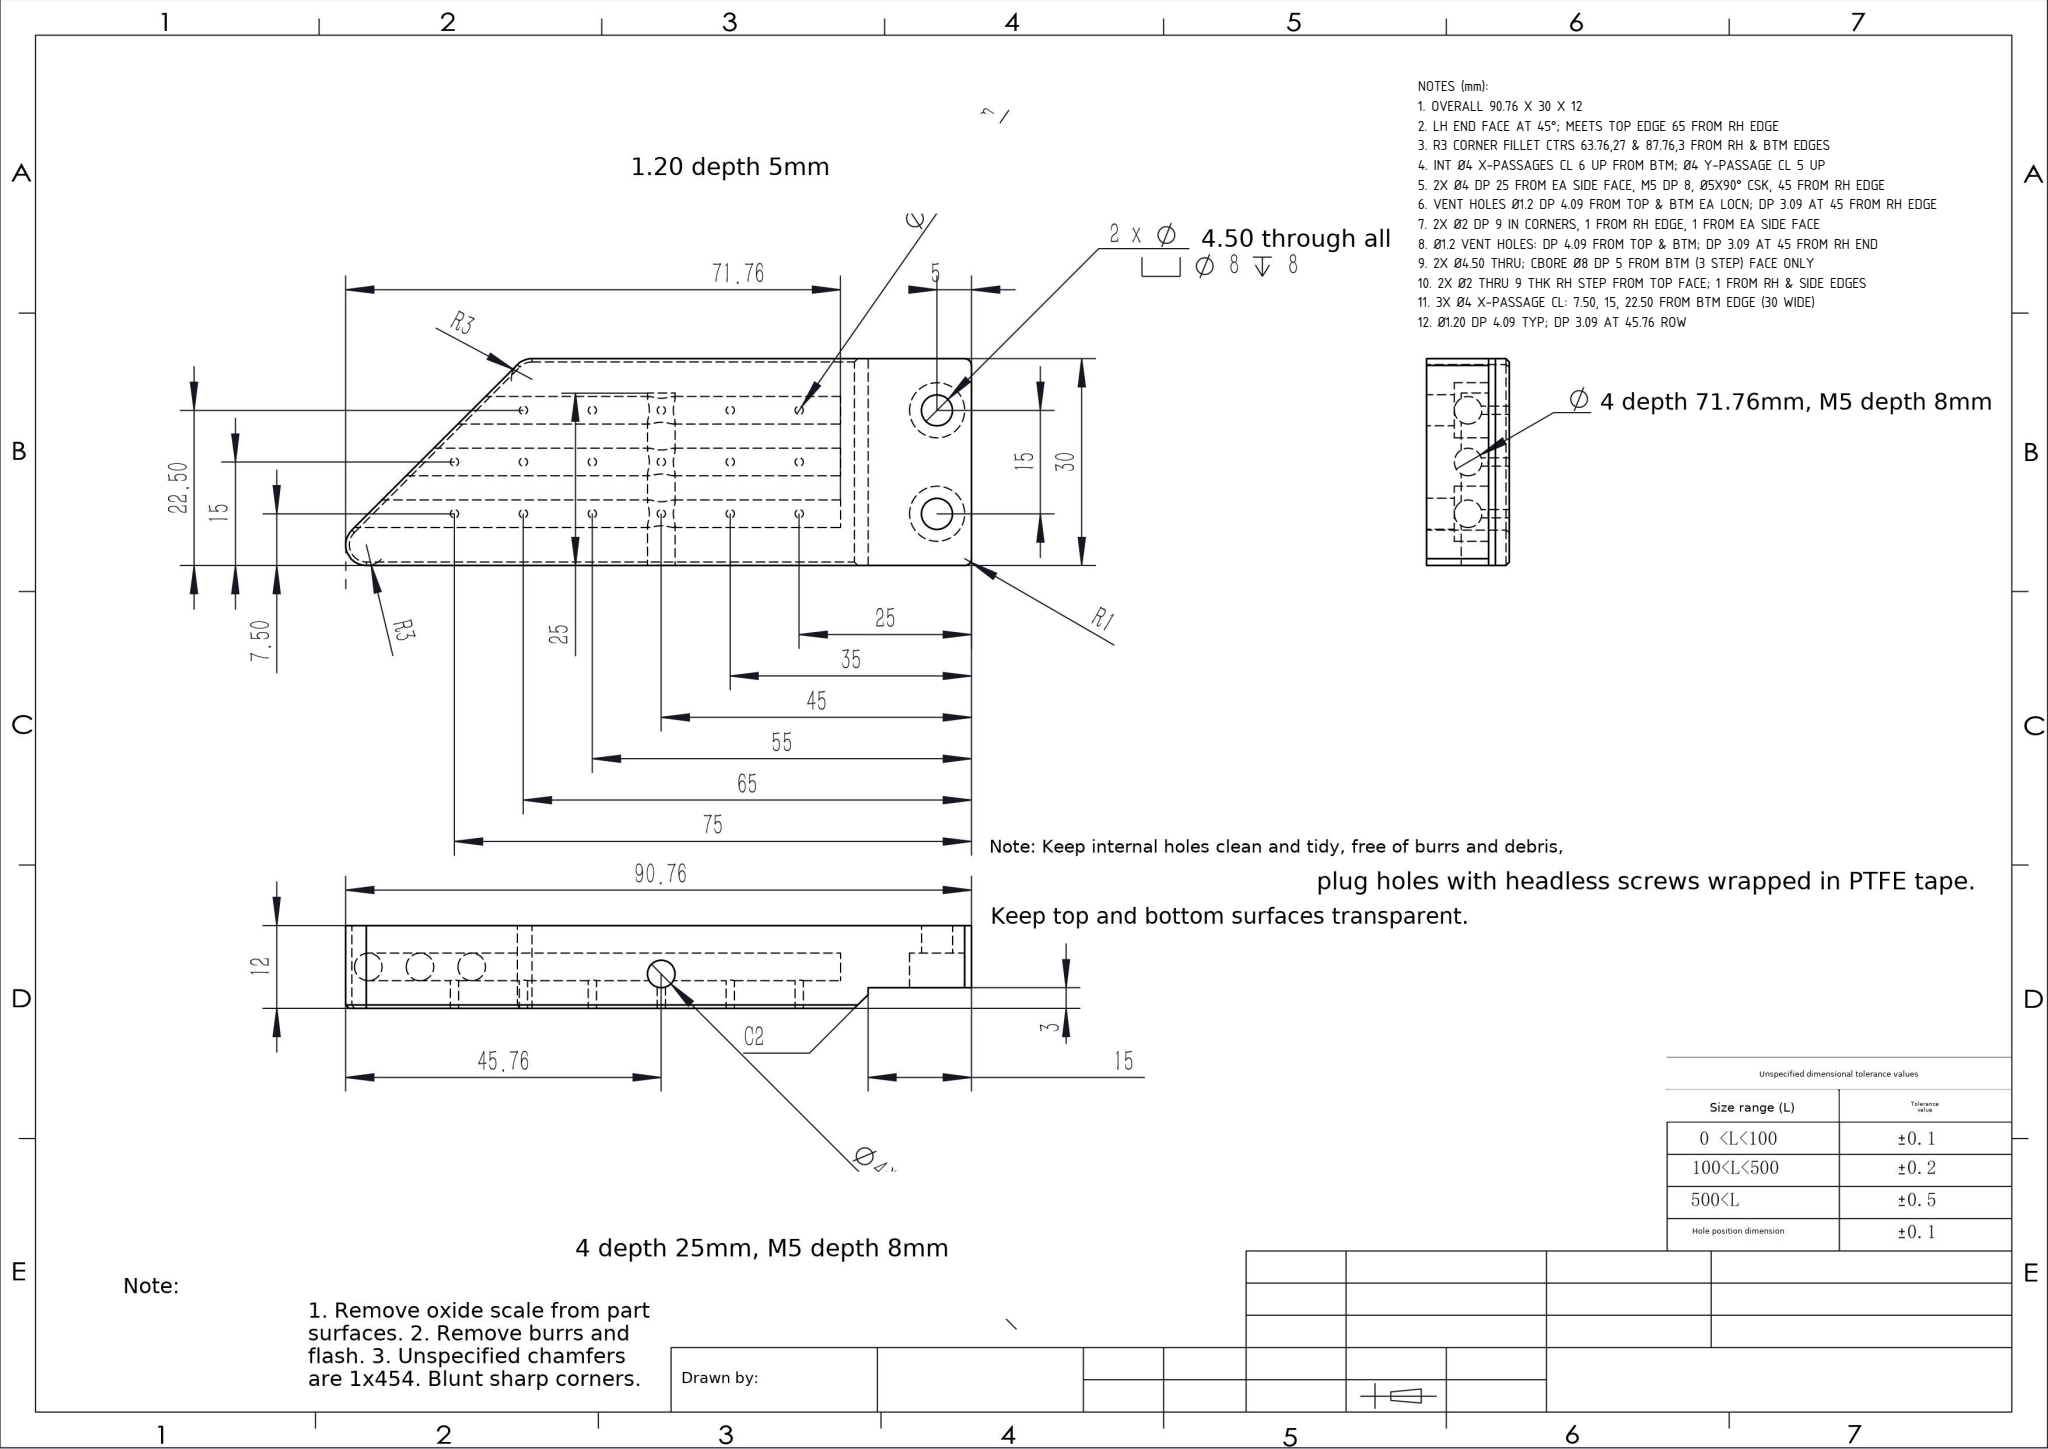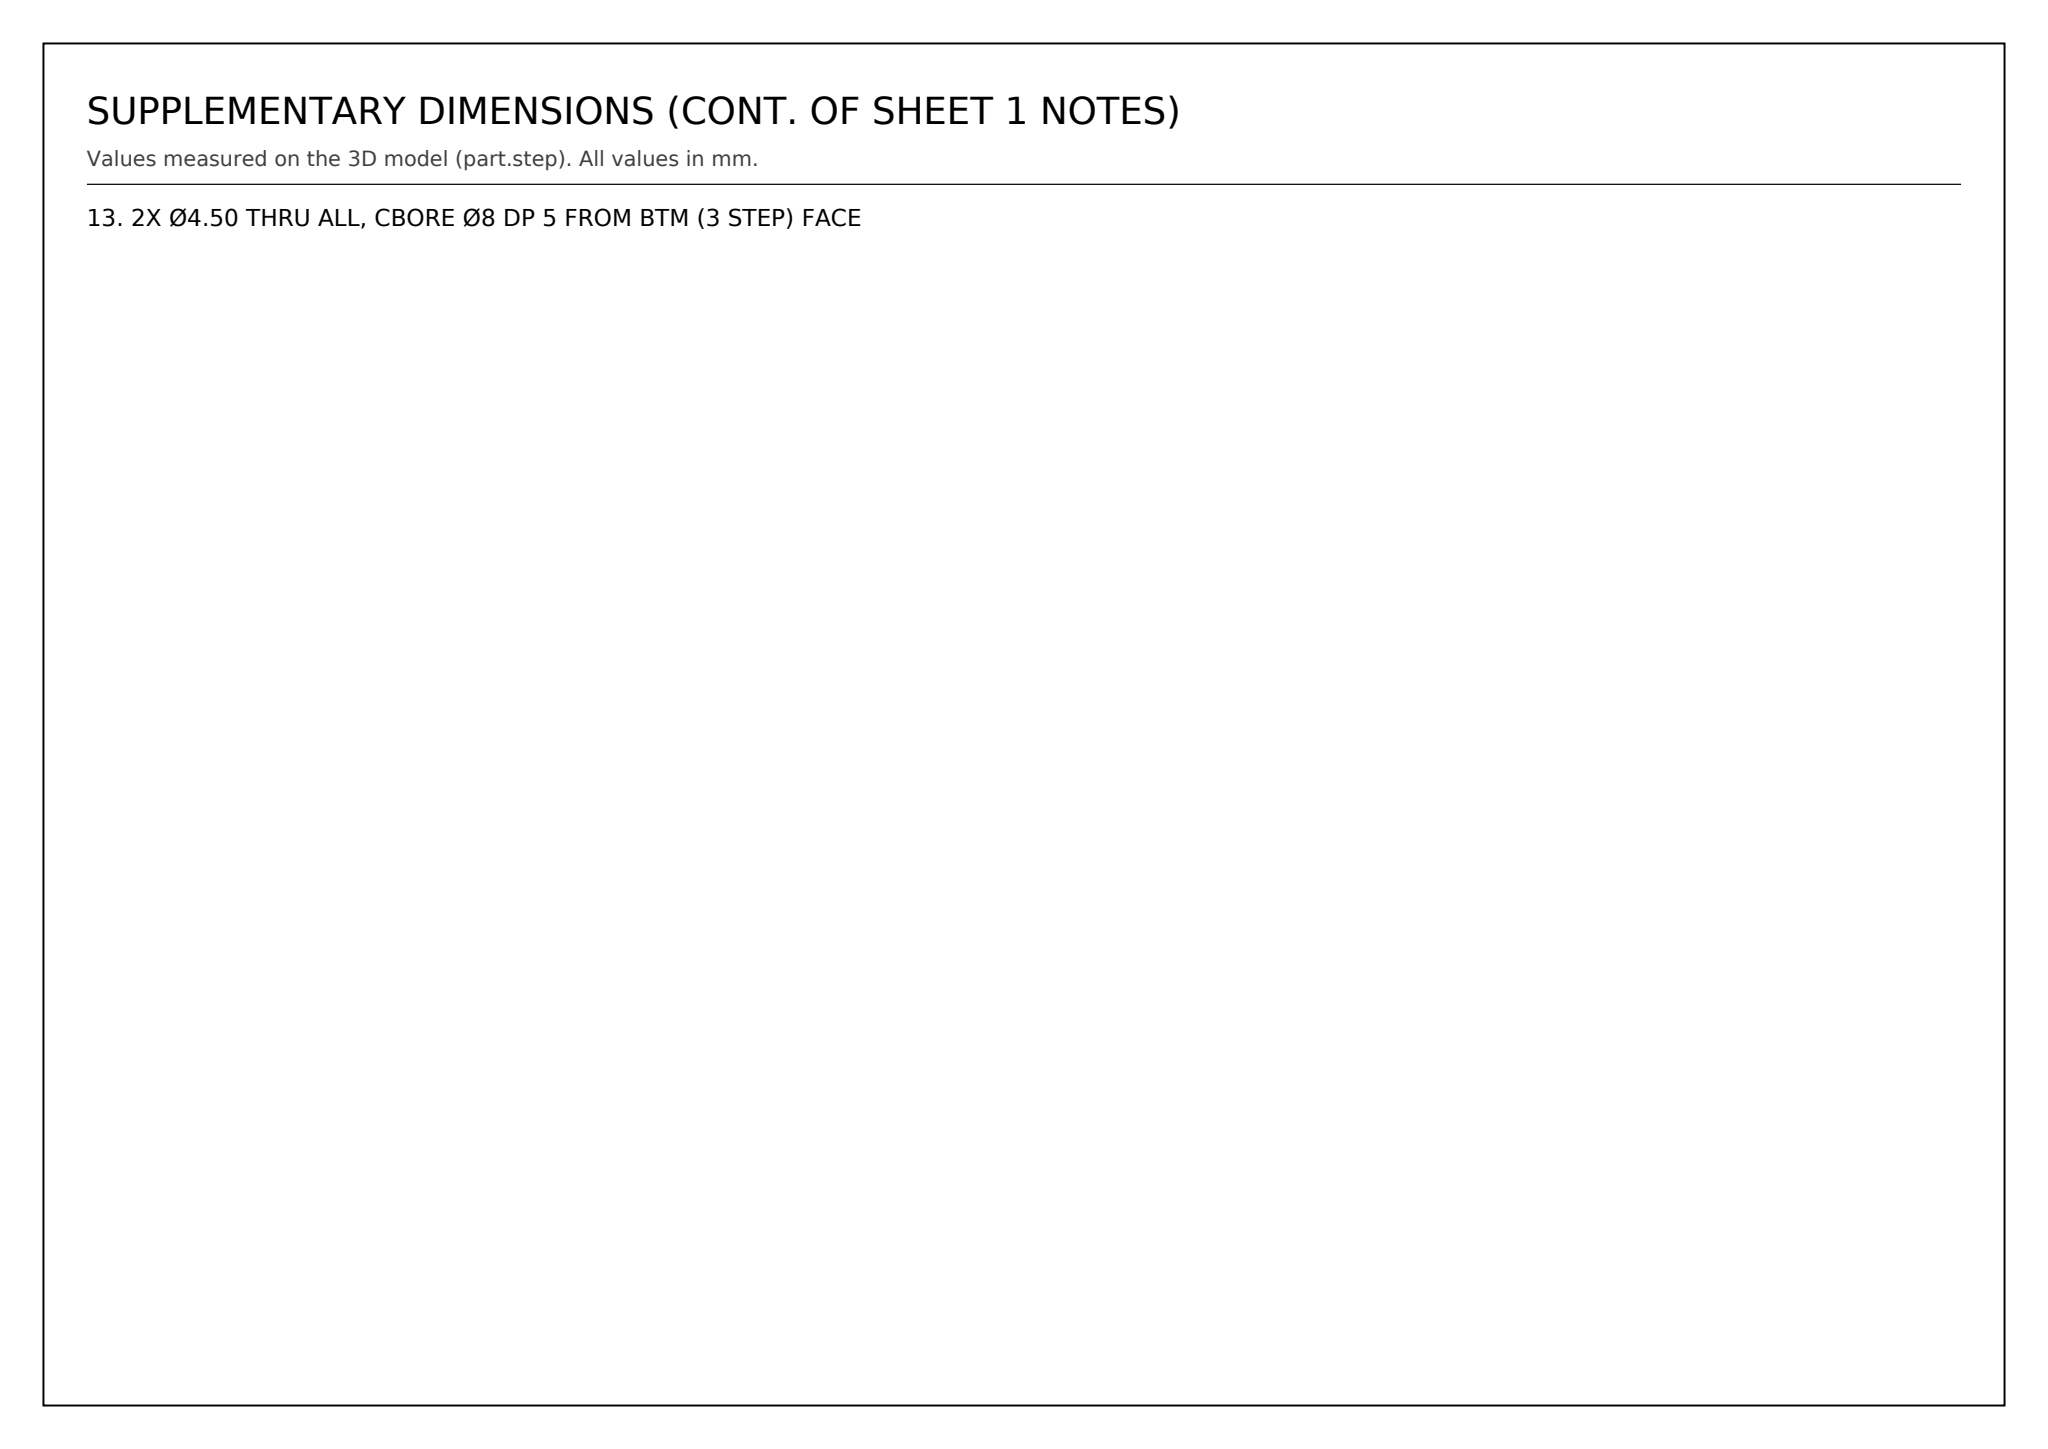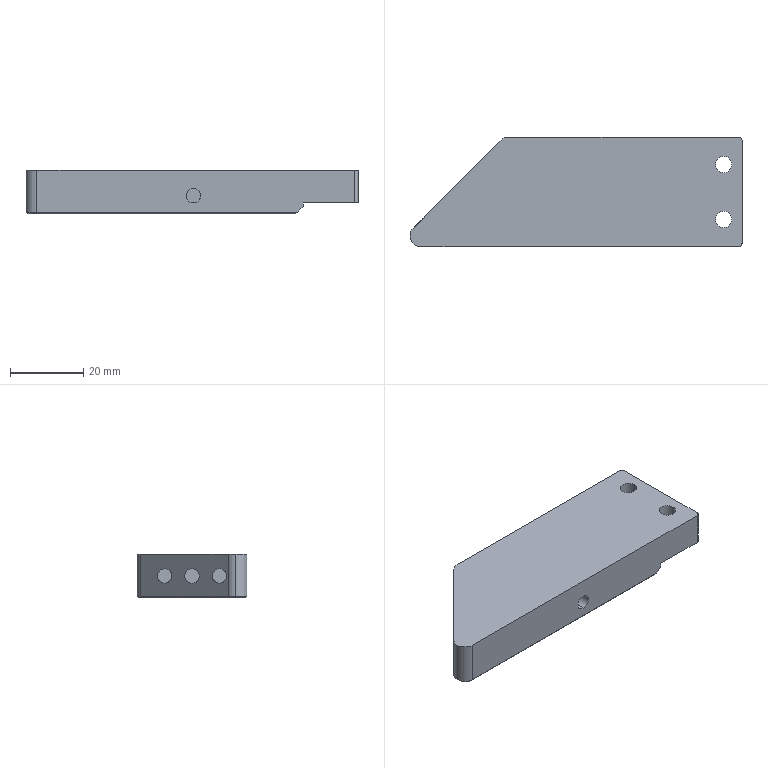Part | SolidWorks | mm | 1 solid | 78 faces | box 90.76 x 30 x 12 mm | volume 24014 mm3 | cylinder 58 | plane 18 | cone 2 | commonest cylinder face diameters 1.2 x34 4 x11 8 x4 4.5 x4 6 x3 2 x2
Drawing notes:
OVERALL 90.76 X 30 X 12 | from the solid: bbox_xyz [90.757, 30.0, 12.0]
LH END FACE AT 45°; MEETS TOP EDGE 65 FROM RH EDGE | from the solid: R3 arc ctrs (3,3) & (27,27) give 45° line; top edge y=30 at x=25.757 = 65 from RH edge x=90.757
R3 CORNER FILLET CTRS 63.76,27 & 87.76,3 FROM RH & BTM EDGES | from the solid: cyl dia 6.0 axis z at (27.0,27.0) and (3.0,3.0); 90.757-27=63.76, 90.757-3=87.76
INT Ø4 X-PASSAGES CL 6 UP FROM BTM; Ø4 Y-PASSAGE CL 5 UP | from the solid: cylinders dia 4 axis x at z=6.0; dia 4 axis y at z=5.0; bbox z=12
2X Ø4 DP 25 FROM EA SIDE FACE, M5 DP 8, Ø5X90° CSK, 45 FROM RH EDGE | from the solid: [4.0,'y',[45.76,null,5.0],25.0,2] with cones[90.0, ref dia 5.0] x2; 90.757-45.76=45
VENT HOLES Ø1.2 DP 4.09 FROM TOP & BTM EA LOCN; DP 3.09 AT 45 FROM RH EDGE | from the solid: dia 1.2 axis z len 4.09 x2 at x=15.76..65.76, y=7.5/15/22.5; len 3.09 at x=45.76
2X Ø2 DP 9 IN CORNERS, 1 FROM RH EDGE, 1 FROM EA SIDE FACE | from the solid: cyl dia 2.0 axis z at (89.76,1.0) & (89.76,29.0), len 9.0; bbox 90.757x30.0
Ø1.2 VENT HOLES: DP 4.09 FROM TOP & BTM; DP 3.09 AT 45 FROM RH END | from the solid: Ø1.2 z-axis cyls L=4.09 (2 ea) at x=15.76/25.76/35.76/55.76/65.76; L=3.09 (2 ea) at x=45.76 i.e. 45 from RH face x=90.76
2X Ø4.50 THRU; CBORE Ø8 DP 5 FROM BTM (3 STEP) FACE ONLY | from the solid: Ø8 z-cyl L=5 from z=3 step face to z=8 plane (2 planes @ z=8), then Ø4.5 L=4 to z=12 top; 5+4=9 = step thk (z 3..12)
2X Ø2 THRU 9 THK RH STEP FROM TOP FACE; 1 FROM RH & SIDE EDGES | from the solid: Ø2 z-cyls L=9 at x=89.76 (1 from x=90.76 edge), y=1.0 & 29.0 (1 from y=0/30); L=9 = local thk z=3..12
3X Ø4 X-PASSAGE CL: 7.50, 15, 22.50 FROM BTM EDGE (30 WIDE) | from the solid: cylinders dia 4 axis x at y=7.5, 15.0, 22.5, z=6.0
Ø1.20 DP 4.09 TYP; DP 3.09 AT 45.76 ROW | from the solid: Ø1.2 z-holes length 4.09, except x=45.76 length 3.09
2X Ø4.50 THRU ALL, CBORE Ø8 DP 5 FROM BTM (3 STEP) FACE | from the solid: Ø4.5 z-holes L=4.0; Ø8 z-cbores L=5.0 at x=85.76, y=7.5 & 22.5
build123d program:
from build123d import *

# Parameters (mm, degrees)
SKETCH1_W                                            = 95
SKETCH1_H                                            = 30
BOSS_EXTRUDE1_DEPTH                                  = 12
HOLE_SIZE_ACCORDING_TO_THE_TYPE_OF_HEXAG_D           = 4.5
HOLE_SIZE_ACCORDING_TO_THE_TYPE_OF_HEXAG_CBORE_D     = 8
HOLE_SIZE_ACCORDING_TO_THE_TYPE_OF_HEXAG_CBORE_DEPTH = 8
SKETCH4_W                                            = 15
SKETCH4_H                                            = 30
CUT_EXTRUDE1_DEPTH                                   = 3
SKETCH5_R                                            = 2
BOSS_EXTRUDE2_DEPTH                                  = 76
SKETCH6_R                                            = 2
CUT_EXTRUDE2_DEPTH                                   = 76
SKETCH7_R                                            = 0.6
CUT_EXTRUDE3_DEPTH                                   = 5
SKETCH8_R                                            = 2
CUT_EXTRUDE4_DEPTH                                   = 25
FILLET2_R                                            = 1
CUT_EXTRUDE5_DEPTH                                   = 52.237
CUT_EXTRUDE5_DEPTH_BACK                              = 52.237
FILLET3_R                                            = 3
CHAMFER1_SIZE                                        = 2
CHAMFER2_SIZE                                        = 0.5


with BuildPart() as part:
    # Sketch1 → Boss-Extrude1 (new body)
    with BuildSketch(Plane.XY):
        Rectangle(SKETCH1_W, SKETCH1_H)
    extrude(amount=BOSS_EXTRUDE1_DEPTH)

    # Hole size according to the type of hexag (through all)
    with Locations(Plane(origin=(0, 0, 0), x_dir=(-1, 0, 0), z_dir=(0, 0, -1))):
        with Locations((-42.5, -7.5), (-42.5, 7.5)):
            CounterBoreHole(HOLE_SIZE_ACCORDING_TO_THE_TYPE_OF_HEXAG_D / 2, HOLE_SIZE_ACCORDING_TO_THE_TYPE_OF_HEXAG_CBORE_D / 2, HOLE_SIZE_ACCORDING_TO_THE_TYPE_OF_HEXAG_CBORE_DEPTH)

    # Sketch4 → Cut-Extrude1 (cut)
    with BuildSketch(Plane(origin=(0, 0, 0), x_dir=(-1, 0, 0), z_dir=(0, 0, -1))):
        with Locations((-40, 0)):
            Rectangle(SKETCH4_W, SKETCH4_H)
    extrude(amount=-CUT_EXTRUDE1_DEPTH, mode=Mode.SUBTRACT)

    # Sketch5 → Boss-Extrude2 (add)
    with BuildSketch(Plane.ZY.offset(47.5)):
        with Locations((6, 0)):
            Circle(SKETCH5_R)
    extrude(amount=-BOSS_EXTRUDE2_DEPTH)

    # Sketch6 → Cut-Extrude2 (cut)
    with BuildSketch(Plane.ZY.offset(47.5)):
        with Locations(Location((6, -7.5, 0), (0, 0, 270))):
            Circle(SKETCH6_R)
        with Locations(Location((6, 0, 0), (0, 0, 270))):
            Circle(SKETCH6_R)
        with Locations(Location((6, 7.5, 0), (0, 0, 270))):
            Circle(SKETCH6_R)
    extrude(amount=-CUT_EXTRUDE2_DEPTH, mode=Mode.SUBTRACT)

    # Sketch7 → Cut-Extrude3 (cut)
    with BuildSketch(Plane(origin=(0, 0, 0), x_dir=(-1, 0, 0), z_dir=(0, 0, -1))):
        with Locations((27.5, 7.5)):
            Circle(SKETCH7_R)
        with Locations((17.5, 7.5)):
            Circle(SKETCH7_R)
        with Locations((7.5, 7.5)):
            Circle(SKETCH7_R)
        with Locations((-2.5, 7.5)):
            Circle(SKETCH7_R)
        with Locations((-12.5, 7.5)):
            Circle(SKETCH7_R)
        with Locations((-22.5, 7.5)):
            Circle(SKETCH7_R)
        with Locations((27.5, 0)):
            Circle(SKETCH7_R)
        with Locations((17.5, 0)):
            Circle(SKETCH7_R)
        with Locations((7.5, 0)):
            Circle(SKETCH7_R)
        with Locations((-2.5, 0)):
            Circle(SKETCH7_R)
        with Locations((-12.5, 0)):
            Circle(SKETCH7_R)
        with Locations((-22.5, 0)):
            Circle(SKETCH7_R)
        with Locations((27.5, -7.5)):
            Circle(SKETCH7_R)
        with Locations((17.5, -7.5)):
            Circle(SKETCH7_R)
        with Locations((7.5, -7.5)):
            Circle(SKETCH7_R)
        with Locations((-2.5, -7.5)):
            Circle(SKETCH7_R)
        with Locations((-12.5, -7.5)):
            Circle(SKETCH7_R)
        with Locations((-22.5, -7.5)):
            Circle(SKETCH7_R)
    extrude(amount=-CUT_EXTRUDE3_DEPTH, mode=Mode.SUBTRACT)

    # Sketch8 → Cut-Extrude4 (cut)
    with BuildSketch(Plane.XZ.offset(15)):
        with Locations(Location((2.5, 5, 0), (0, 0, 270))):
            Circle(SKETCH8_R)
    extrude(amount=-CUT_EXTRUDE4_DEPTH, mode=Mode.SUBTRACT)

    # Fillet2
    fillet2_edges = [part.edges().sort_by_distance(p)[0] for p in [
        (47.5, -15, 7.5),
        (47.5, 15, 7.5),
    ]]
    fillet(fillet2_edges, radius=FILLET2_R)

    # Sketch9 → Cut-Extrude5 (cut, two sides: drawn at the far end of the back side and taken through both)
    with BuildSketch(Plane(origin=(0, 0, 0), x_dir=(-1, 0, 0), z_dir=(0, 0, -1)).offset(-CUT_EXTRUDE5_DEPTH_BACK)):
        Polygon((195.461, -162.961), (47.5, -15), (17.5, 15), (-130.461, 162.961), (165.461, 458.883), (491.383, 132.961), align=None)
    extrude(amount=CUT_EXTRUDE5_DEPTH + CUT_EXTRUDE5_DEPTH_BACK, mode=Mode.SUBTRACT)

    # Fillet3
    fillet3_edges = [part.edges().sort_by_distance(p)[0] for p in [
        (-17.5, 15, 6),
        (-47.5, -15, 6),
    ]]
    fillet(fillet3_edges, radius=FILLET3_R)

    # Chamfer1
    chamfer1_edges = [part.edges().sort_by_distance(p)[0] for p in [
        (32.5, 0, 0),
    ]]
    chamfer(chamfer1_edges, length=CHAMFER1_SIZE)

    # Chamfer2
    chamfer2_edges = [part.edges().sort_by_distance(p)[0] for p in [
        (-4.879, -15, 0),
        (-30.379, 2.121, 0),
        (-17.405, 14.772, 0),
        (-43.029, -13.148, 0),
        (7.121, 15, 0),
    ]]
    chamfer(chamfer2_edges, length=CHAMFER2_SIZE)


solid = part.part